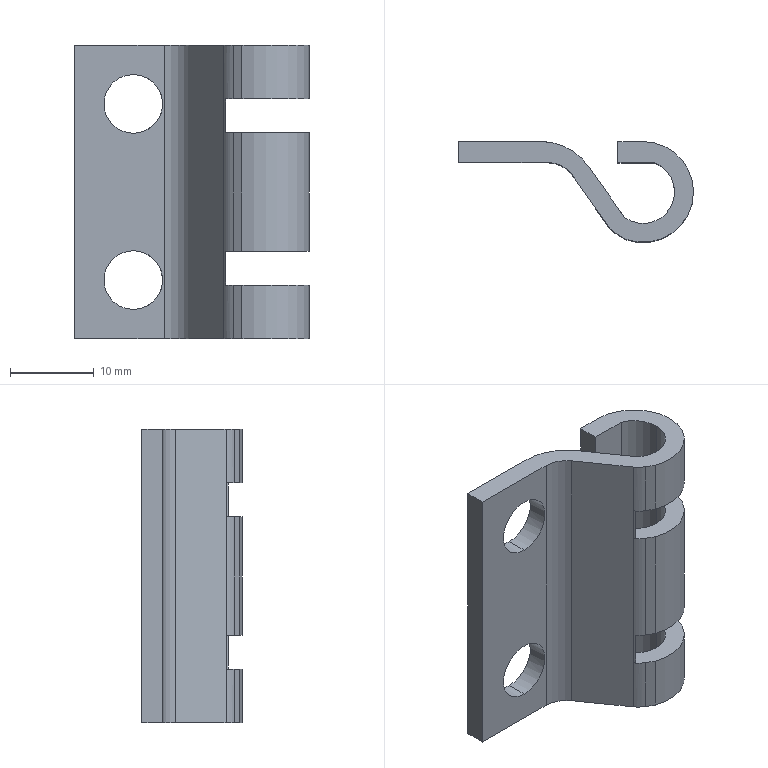Component | SolidWorks | OuterDoorAssembly1-1_HHL011-1RittalHingeMiddleShaftSleeve-2 | 1 solid | 44 faces | volume 2990 mm3 | plane 25 | cylinder 19 | commonest cylinder face diameters 7 x6 11.998 x6 7.5 x6 14 x1